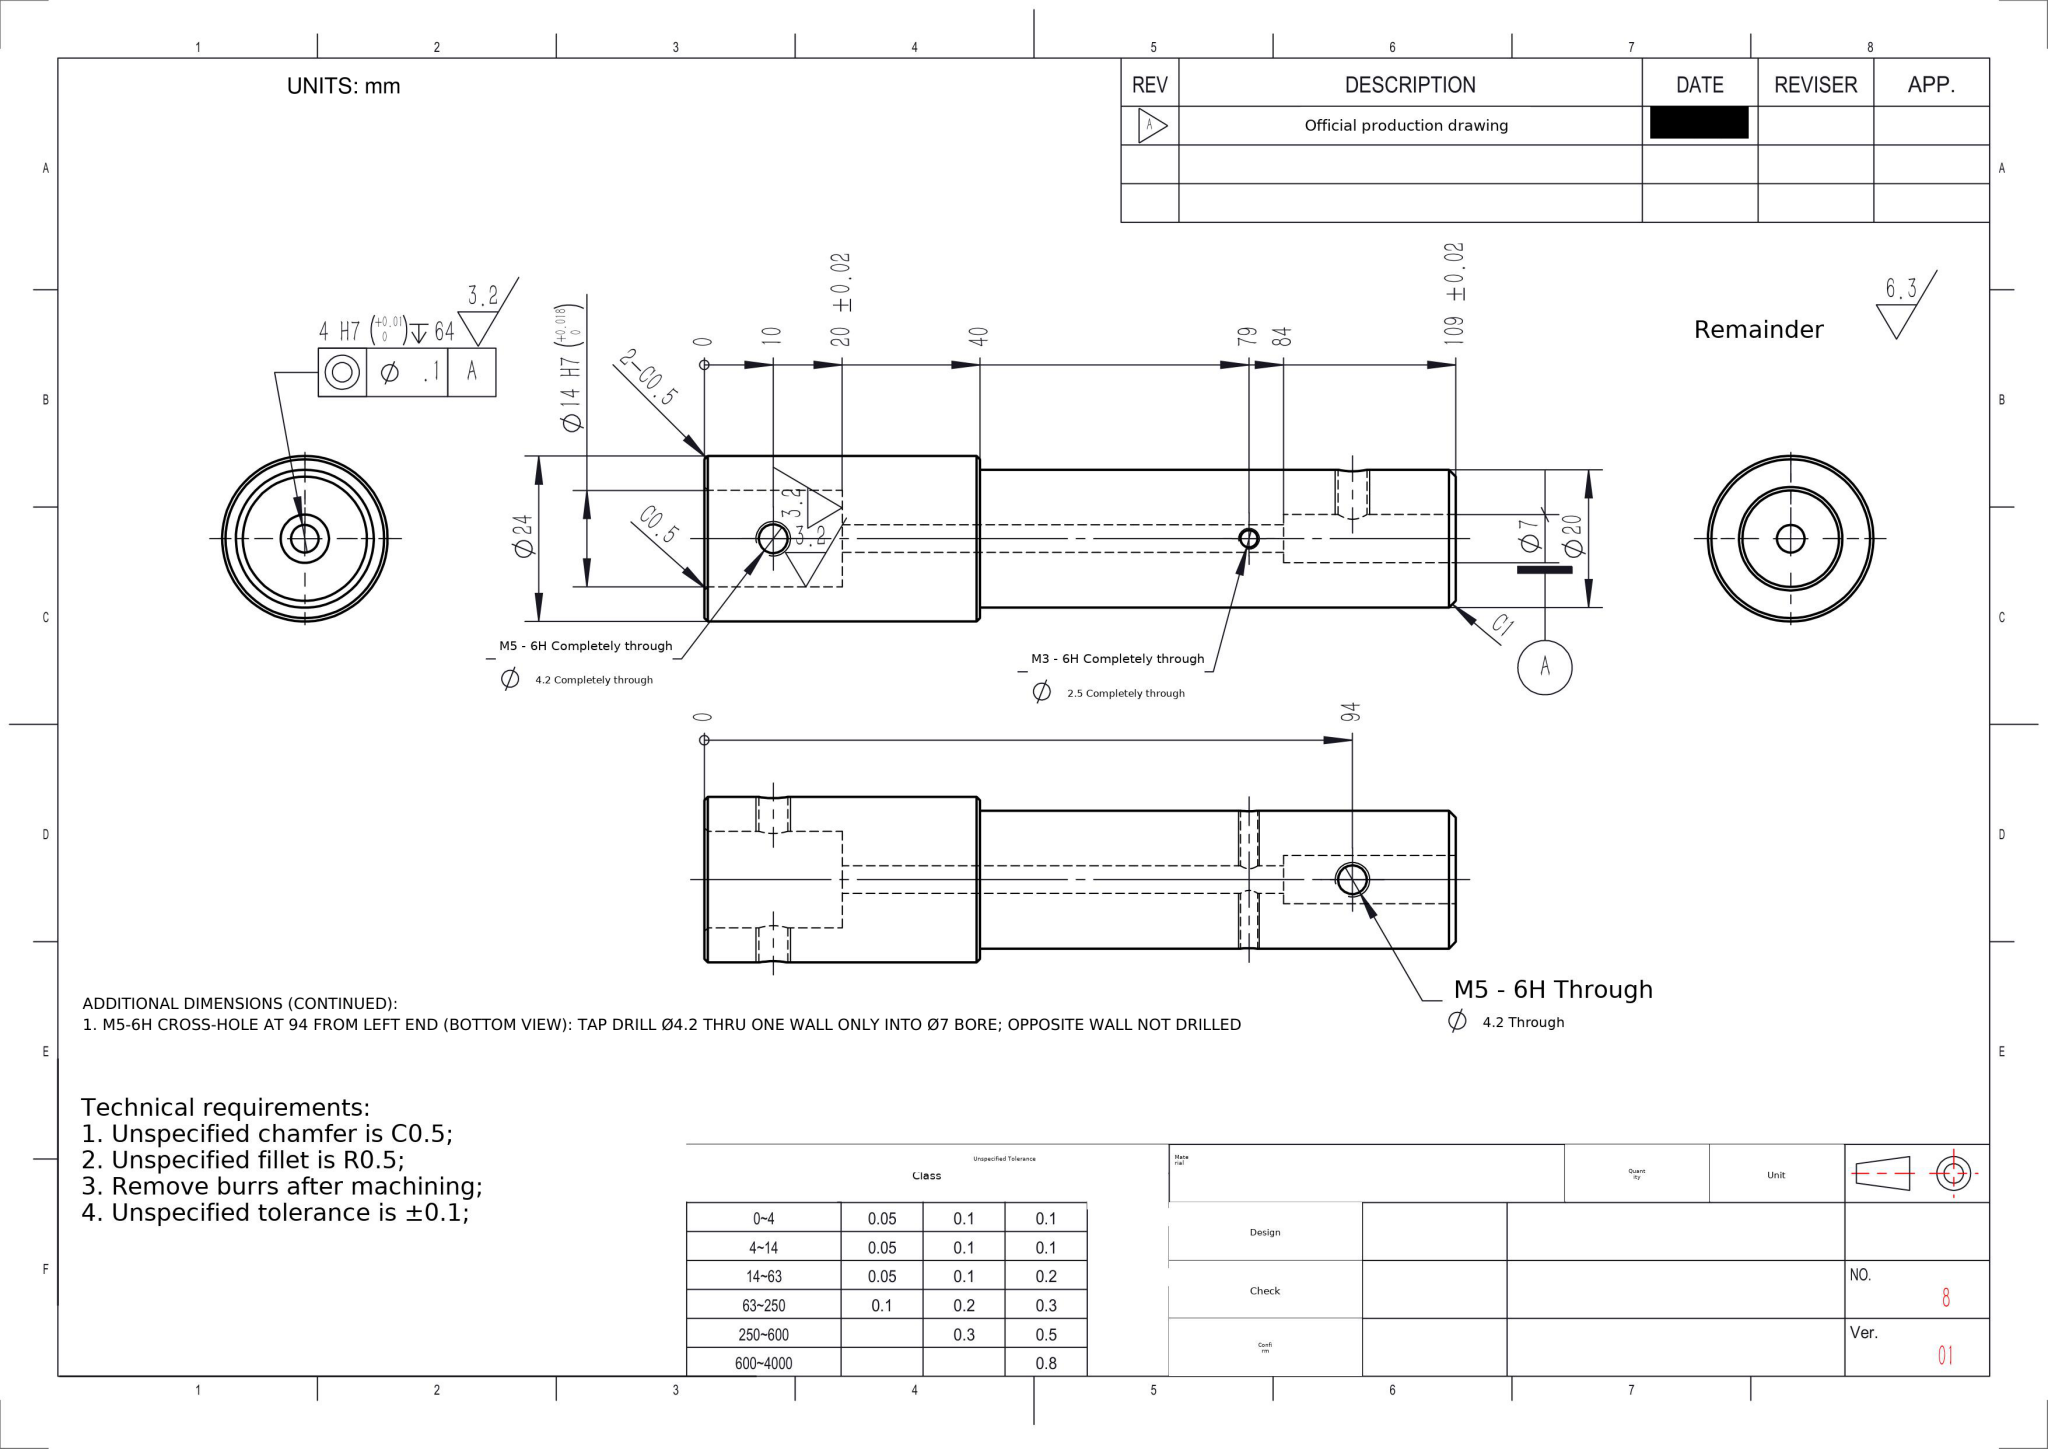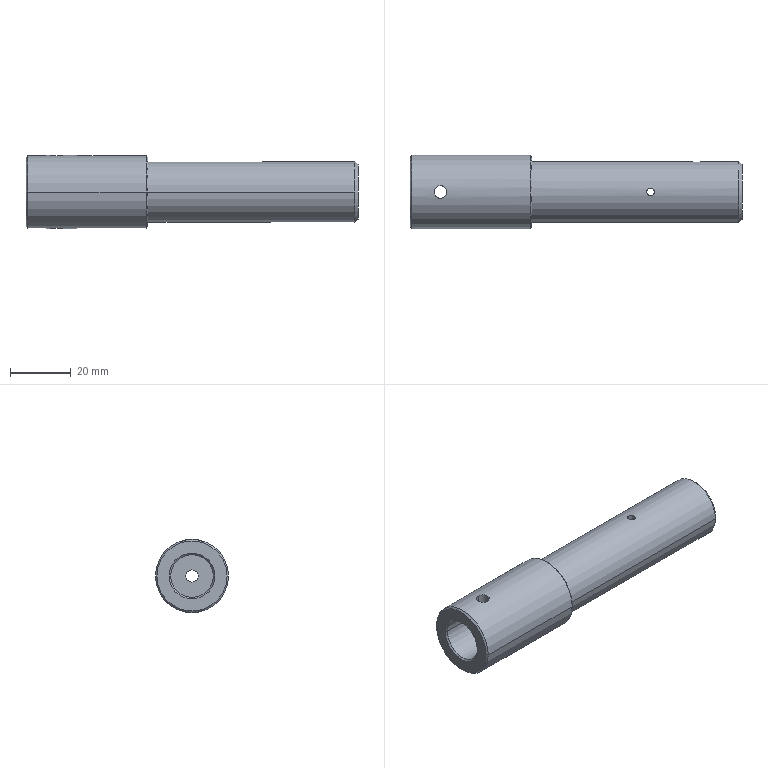Part | NX | mm | 1 solid | 33 faces | box 109 x 24 x 24 mm | volume 34562 mm3 | cylinder 20 | cone 8 | plane 5 | commonest cylinder face diameters 4.2 x6 2.5 x4 4 x2 7 x2 14 x2 20 x2 24 x2